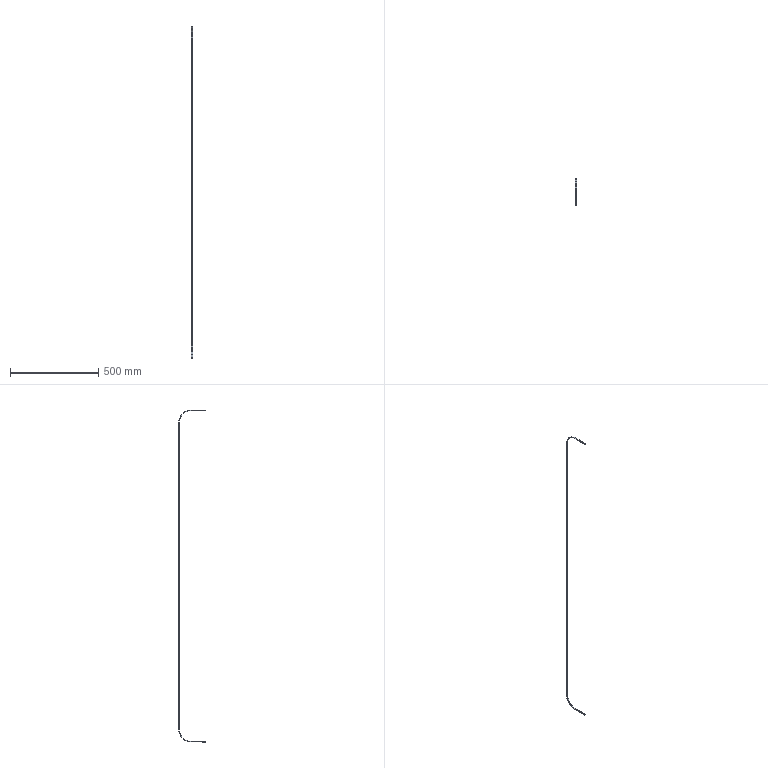Component | SolidWorks | TopHousingAssembly-1_Sealant-2 | 1 solid | 22 faces | box 6 x 149.5 x 1881 mm | volume 38081 mm3 | plane 18 | cylinder 4 | commonest cylinder face diameters 139 x2 133 x2
STEP:
#1=CARTESIAN_POINT('',(43.307,96.791,2.618));
#2=VERTEX_POINT('',#1);
#3=CARTESIAN_POINT('',(43.307,96.909,2.618));
#4=VERTEX_POINT('',#3);
#5=CARTESIAN_POINT('',(43.307,96.909,2.618));
#6=DIRECTION('',(0.,1.,0.));
#7=VECTOR('',#6,39.37);
#8=LINE('',#5,#7);
#9=EDGE_CURVE('',#2,#4,#8,.T.);
#10=ORIENTED_EDGE('',*,*,#9,.F.);
#11=CARTESIAN_POINT('',(43.307,96.791,71.201));
#12=VERTEX_POINT('',#11);
#13=CARTESIAN_POINT('',(43.307,96.791,36.909));
#14=DIRECTION('',(0.,0.,-1.));
#15=VECTOR('',#14,39.37);
#16=LINE('',#13,#15);
#17=EDGE_CURVE('',#12,#2,#16,.T.);
#18=ORIENTED_EDGE('',*,*,#17,.F.);
#19=CARTESIAN_POINT('',(43.307,96.909,71.201));
#20=VERTEX_POINT('',#19);
#21=CARTESIAN_POINT('',(43.307,96.909,71.201));
#22=DIRECTION('',(0.,1.,0.));
#23=VECTOR('',#22,39.37);
#24=LINE('',#21,#23);
#25=EDGE_CURVE('',#12,#20,#24,.T.);
#26=ORIENTED_EDGE('',*,*,#25,.T.);
#27=CARTESIAN_POINT('',(43.307,96.909,71.201));
#28=DIRECTION('',(-0.,0.,-1.));
#29=VECTOR('',#28,39.37);
#30=LINE('',#27,#29);
#31=EDGE_CURVE('',#20,#4,#30,.T.);
#32=ORIENTED_EDGE('',*,*,#31,.T.);
#33=EDGE_LOOP('',(#10,#18,#26,#32));
#34=FACE_OUTER_BOUND('',#33,.T.);
#35=CARTESIAN_POINT('',(43.307,96.909,71.201));
#36=DIRECTION('',(-1.,0.,0.));
#37=DIRECTION('',(-0.,0.,-1.));
#38=AXIS2_PLACEMENT_3D('',#35,#36,#37);
#39=PLANE('',#38);
#40=ADVANCED_FACE('',(#34),#39,.T.);
#41=CARTESIAN_POINT('',(43.543,96.791,71.201));
#42=VERTEX_POINT('',#41);
#43=CARTESIAN_POINT('',(43.543,96.909,71.201));
#44=VERTEX_POINT('',#43);
#45=CARTESIAN_POINT('',(43.543,96.909,71.201));
#46=DIRECTION('',(0.,1.,0.));
#47=VECTOR('',#46,39.37);
#48=LINE('',#45,#47);
#49=EDGE_CURVE('',#42,#44,#48,.T.);
#50=ORIENTED_EDGE('',*,*,#49,.F.);
#51=CARTESIAN_POINT('',(43.543,96.791,2.618));
#52=VERTEX_POINT('',#51);
#53=CARTESIAN_POINT('',(43.543,96.791,36.909));
#54=DIRECTION('',(0.,0.,-1.));
#55=VECTOR('',#54,39.37);
#56=LINE('',#53,#55);
#57=EDGE_CURVE('',#42,#52,#56,.T.);
#58=ORIENTED_EDGE('',*,*,#57,.T.);
#59=CARTESIAN_POINT('',(43.543,96.909,2.618));
#60=VERTEX_POINT('',#59);
#61=CARTESIAN_POINT('',(43.543,96.909,2.618));
#62=DIRECTION('',(0.,1.,0.));
#63=VECTOR('',#62,39.37);
#64=LINE('',#61,#63);
#65=EDGE_CURVE('',#52,#60,#64,.T.);
#66=ORIENTED_EDGE('',*,*,#65,.T.);
#67=CARTESIAN_POINT('',(43.543,96.909,71.201));
#68=DIRECTION('',(-0.,0.,-1.));
#69=VECTOR('',#68,39.37);
#70=LINE('',#67,#69);
#71=EDGE_CURVE('',#44,#60,#70,.T.);
#72=ORIENTED_EDGE('',*,*,#71,.F.);
#73=EDGE_LOOP('',(#50,#58,#66,#72));
#74=FACE_OUTER_BOUND('',#73,.T.);
#75=CARTESIAN_POINT('',(43.543,96.909,71.201));
#76=DIRECTION('',(-1.,0.,0.));
#77=DIRECTION('',(-0.,0.,-1.));
#78=AXIS2_PLACEMENT_3D('',#75,#76,#77);
#79=PLANE('',#78);
#80=ADVANCED_FACE('',(#74),#79,.F.);
#81=ORIENTED_EDGE('',*,*,#71,.T.);
#82=CARTESIAN_POINT('',(43.307,96.909,2.618));
#83=DIRECTION('',(1.,0.,0.));
#84=VECTOR('',#83,39.37);
#85=LINE('',#82,#84);
#86=EDGE_CURVE('',#4,#60,#85,.T.);
#87=ORIENTED_EDGE('',*,*,#86,.F.);
#88=ORIENTED_EDGE('',*,*,#31,.F.);
#89=CARTESIAN_POINT('',(43.543,96.909,71.201));
#90=DIRECTION('',(-1.,0.,0.));
#91=VECTOR('',#90,39.37);
#92=LINE('',#89,#91);
#93=EDGE_CURVE('',#44,#20,#92,.T.);
#94=ORIENTED_EDGE('',*,*,#93,.F.);
#95=EDGE_LOOP('',(#81,#87,#88,#94));
#96=FACE_OUTER_BOUND('',#95,.T.);
#97=CARTESIAN_POINT('',(43.425,96.909,36.909));
#98=DIRECTION('',(0.,-1.,0.));
#99=DIRECTION('',(-1.,0.,0.));
#100=AXIS2_PLACEMENT_3D('',#97,#98,#99);
#101=PLANE('',#100);
#102=ADVANCED_FACE('',(#96),#101,.F.);
#103=ORIENTED_EDGE('',*,*,#57,.F.);
#104=CARTESIAN_POINT('',(43.425,96.791,71.201));
#105=DIRECTION('',(-1.,0.,0.));
#106=VECTOR('',#105,39.37);
#107=LINE('',#104,#106);
#108=EDGE_CURVE('',#42,#12,#107,.T.);
#109=ORIENTED_EDGE('',*,*,#108,.T.);
#110=ORIENTED_EDGE('',*,*,#17,.T.);
#111=CARTESIAN_POINT('',(43.425,96.791,2.618));
#112=DIRECTION('',(1.,0.,0.));
#113=VECTOR('',#112,39.37);
#114=LINE('',#111,#113);
#115=EDGE_CURVE('',#2,#52,#114,.T.);
#116=ORIENTED_EDGE('',*,*,#115,.T.);
#117=EDGE_LOOP('',(#103,#109,#110,#116));
#118=FACE_OUTER_BOUND('',#117,.T.);
#119=CARTESIAN_POINT('',(43.425,96.791,36.909));
#120=DIRECTION('',(0.,-1.,0.));
#121=DIRECTION('',(-1.,0.,0.));
#122=AXIS2_PLACEMENT_3D('',#119,#120,#121);
#123=PLANE('',#122);
#124=ADVANCED_FACE('',(#118),#123,.T.);
#125=CARTESIAN_POINT('',(43.543,94.173,73.819));
#126=VERTEX_POINT('',#125);
#127=CARTESIAN_POINT('',(43.543,94.173,73.937));
#128=VERTEX_POINT('',#127);
#129=CARTESIAN_POINT('',(43.543,94.173,73.937));
#130=DIRECTION('',(0.,0.,1.));
#131=VECTOR('',#130,39.37);
#132=LINE('',#129,#131);
#133=EDGE_CURVE('',#126,#128,#132,.T.);
#134=ORIENTED_EDGE('',*,*,#133,.F.);
#135=CARTESIAN_POINT('',(43.543,94.173,71.201));
#136=DIRECTION('',(1.,0.,0.));
#137=DIRECTION('',(0.,-0.,1.));
#138=AXIS2_PLACEMENT_3D('',#135,#136,#137);
#139=CIRCLE('',#138,2.618);
#140=EDGE_CURVE('',#42,#126,#139,.T.);
#141=ORIENTED_EDGE('',*,*,#140,.F.);
#142=ORIENTED_EDGE('',*,*,#49,.T.);
#143=CARTESIAN_POINT('',(43.543,94.173,71.201));
#144=DIRECTION('',(1.,0.,0.));
#145=DIRECTION('',(0.,-0.,1.));
#146=AXIS2_PLACEMENT_3D('',#143,#144,#145);
#147=CIRCLE('',#146,2.736);
#148=EDGE_CURVE('',#44,#128,#147,.T.);
#149=ORIENTED_EDGE('',*,*,#148,.T.);
#150=EDGE_LOOP('',(#134,#141,#142,#149));
#151=FACE_OUTER_BOUND('',#150,.T.);
#152=CARTESIAN_POINT('',(43.543,94.173,71.201));
#153=DIRECTION('',(1.,0.,0.));
#154=DIRECTION('',(0.,0.,-1.));
#155=AXIS2_PLACEMENT_3D('',#152,#153,#154);
#156=PLANE('',#155);
#157=ADVANCED_FACE('',(#151),#156,.T.);
#158=CARTESIAN_POINT('',(43.307,94.173,73.819));
#159=VERTEX_POINT('',#158);
#160=CARTESIAN_POINT('',(43.307,94.173,71.201));
#161=DIRECTION('',(-1.,0.,0.));
#162=DIRECTION('',(0.,0.,1.));
#163=AXIS2_PLACEMENT_3D('',#160,#161,#162);
#164=CIRCLE('',#163,2.618);
#165=EDGE_CURVE('',#159,#12,#164,.T.);
#166=ORIENTED_EDGE('',*,*,#165,.F.);
#167=CARTESIAN_POINT('',(43.307,94.173,73.937));
#168=VERTEX_POINT('',#167);
#169=CARTESIAN_POINT('',(43.307,94.173,73.819));
#170=DIRECTION('',(0.,0.,1.));
#171=VECTOR('',#170,39.37);
#172=LINE('',#169,#171);
#173=EDGE_CURVE('',#159,#168,#172,.T.);
#174=ORIENTED_EDGE('',*,*,#173,.T.);
#175=CARTESIAN_POINT('',(43.307,94.173,71.201));
#176=DIRECTION('',(-1.,0.,0.));
#177=DIRECTION('',(0.,0.,1.));
#178=AXIS2_PLACEMENT_3D('',#175,#176,#177);
#179=CIRCLE('',#178,2.736);
#180=EDGE_CURVE('',#168,#20,#179,.T.);
#181=ORIENTED_EDGE('',*,*,#180,.T.);
#182=ORIENTED_EDGE('',*,*,#25,.F.);
#183=EDGE_LOOP('',(#166,#174,#181,#182));
#184=FACE_OUTER_BOUND('',#183,.T.);
#185=CARTESIAN_POINT('',(43.307,94.173,71.201));
#186=DIRECTION('',(1.,0.,0.));
#187=DIRECTION('',(0.,0.,-1.));
#188=AXIS2_PLACEMENT_3D('',#185,#186,#187);
#189=PLANE('',#188);
#190=ADVANCED_FACE('',(#184),#189,.F.);
#191=ORIENTED_EDGE('',*,*,#93,.T.);
#192=ORIENTED_EDGE('',*,*,#180,.F.);
#193=CARTESIAN_POINT('',(43.543,94.173,73.937));
#194=DIRECTION('',(1.,0.,0.));
#195=VECTOR('',#194,39.37);
#196=LINE('',#193,#195);
#197=EDGE_CURVE('',#168,#128,#196,.T.);
#198=ORIENTED_EDGE('',*,*,#197,.T.);
#199=ORIENTED_EDGE('',*,*,#148,.F.);
#200=EDGE_LOOP('',(#191,#192,#198,#199));
#201=FACE_OUTER_BOUND('',#200,.T.);
#202=CARTESIAN_POINT('',(43.307,94.173,71.201));
#203=DIRECTION('',(-1.,0.,0.));
#204=DIRECTION('',(0.,0.,1.));
#205=AXIS2_PLACEMENT_3D('',#202,#203,#204);
#206=CYLINDRICAL_SURFACE('',#205,2.736);
#207=ADVANCED_FACE('',(#201),#206,.T.);
#208=ORIENTED_EDGE('',*,*,#108,.F.);
#209=ORIENTED_EDGE('',*,*,#140,.T.);
#210=CARTESIAN_POINT('',(43.543,94.173,73.819));
#211=DIRECTION('',(-1.,0.,0.));
#212=VECTOR('',#211,39.37);
#213=LINE('',#210,#212);
#214=EDGE_CURVE('',#126,#159,#213,.T.);
#215=ORIENTED_EDGE('',*,*,#214,.T.);
#216=ORIENTED_EDGE('',*,*,#165,.T.);
#217=EDGE_LOOP('',(#208,#209,#215,#216));
#218=FACE_OUTER_BOUND('',#217,.T.);
#219=CARTESIAN_POINT('',(43.307,94.173,71.201));
#220=DIRECTION('',(-1.,0.,0.));
#221=DIRECTION('',(0.,0.,1.));
#222=AXIS2_PLACEMENT_3D('',#219,#220,#221);
#223=CYLINDRICAL_SURFACE('',#222,2.618);
#224=ADVANCED_FACE('',(#218),#223,.F.);
#225=ORIENTED_EDGE('',*,*,#133,.T.);
#226=CARTESIAN_POINT('',(43.543,91.024,73.937));
#227=VERTEX_POINT('',#226);
#228=CARTESIAN_POINT('',(43.543,96.791,73.937));
#229=DIRECTION('',(0.,1.,-0.));
#230=VECTOR('',#229,39.37);
#231=LINE('',#228,#230);
#232=EDGE_CURVE('',#227,#128,#231,.T.);
#233=ORIENTED_EDGE('',*,*,#232,.F.);
#234=CARTESIAN_POINT('',(43.543,91.024,73.819));
#235=VERTEX_POINT('',#234);
#236=CARTESIAN_POINT('',(43.543,91.024,73.937));
#237=DIRECTION('',(0.,-0.,-1.));
#238=VECTOR('',#237,39.37);
#239=LINE('',#236,#238);
#240=EDGE_CURVE('',#227,#235,#239,.T.);
#241=ORIENTED_EDGE('',*,*,#240,.T.);
#242=CARTESIAN_POINT('',(43.543,96.791,73.819));
#243=DIRECTION('',(0.,1.,-0.));
#244=VECTOR('',#243,39.37);
#245=LINE('',#242,#244);
#246=EDGE_CURVE('',#235,#126,#245,.T.);
#247=ORIENTED_EDGE('',*,*,#246,.T.);
#248=EDGE_LOOP('',(#225,#233,#241,#247));
#249=FACE_OUTER_BOUND('',#248,.T.);
#250=CARTESIAN_POINT('',(43.543,96.791,73.937));
#251=DIRECTION('',(-1.,0.,0.));
#252=DIRECTION('',(0.,0.,1.));
#253=AXIS2_PLACEMENT_3D('',#250,#251,#252);
#254=PLANE('',#253);
#255=ADVANCED_FACE('',(#249),#254,.F.);
#256=ORIENTED_EDGE('',*,*,#173,.F.);
#257=CARTESIAN_POINT('',(43.307,91.024,73.819));
#258=VERTEX_POINT('',#257);
#259=CARTESIAN_POINT('',(43.307,91.024,73.819));
#260=DIRECTION('',(0.,-1.,0.));
#261=VECTOR('',#260,39.37);
#262=LINE('',#259,#261);
#263=EDGE_CURVE('',#159,#258,#262,.T.);
#264=ORIENTED_EDGE('',*,*,#263,.T.);
#265=CARTESIAN_POINT('',(43.307,91.024,73.937));
#266=VERTEX_POINT('',#265);
#267=CARTESIAN_POINT('',(43.307,91.024,73.937));
#268=DIRECTION('',(0.,-0.,-1.));
#269=VECTOR('',#268,39.37);
#270=LINE('',#267,#269);
#271=EDGE_CURVE('',#266,#258,#270,.T.);
#272=ORIENTED_EDGE('',*,*,#271,.F.);
#273=CARTESIAN_POINT('',(43.307,96.791,73.937));
#274=DIRECTION('',(0.,-1.,0.));
#275=VECTOR('',#274,39.37);
#276=LINE('',#273,#275);
#277=EDGE_CURVE('',#168,#266,#276,.T.);
#278=ORIENTED_EDGE('',*,*,#277,.F.);
#279=EDGE_LOOP('',(#256,#264,#272,#278));
#280=FACE_OUTER_BOUND('',#279,.T.);
#281=CARTESIAN_POINT('',(43.307,91.024,73.937));
#282=DIRECTION('',(1.,0.,0.));
#283=DIRECTION('',(0.,0.,-1.));
#284=AXIS2_PLACEMENT_3D('',#281,#282,#283);
#285=PLANE('',#284);
#286=ADVANCED_FACE('',(#280),#285,.F.);
#287=ORIENTED_EDGE('',*,*,#197,.F.);
#288=ORIENTED_EDGE('',*,*,#277,.T.);
#289=CARTESIAN_POINT('',(43.425,91.024,73.937));
#290=DIRECTION('',(1.,0.,0.));
#291=VECTOR('',#290,39.37);
#292=LINE('',#289,#291);
#293=EDGE_CURVE('',#266,#227,#292,.T.);
#294=ORIENTED_EDGE('',*,*,#293,.T.);
#295=ORIENTED_EDGE('',*,*,#232,.T.);
#296=EDGE_LOOP('',(#287,#288,#294,#295));
#297=FACE_OUTER_BOUND('',#296,.T.);
#298=CARTESIAN_POINT('',(43.425,96.791,73.937));
#299=DIRECTION('',(0.,-0.,-1.));
#300=DIRECTION('',(0.,1.,-0.));
#301=AXIS2_PLACEMENT_3D('',#298,#299,#300);
#302=PLANE('',#301);
#303=ADVANCED_FACE('',(#297),#302,.F.);
#304=ORIENTED_EDGE('',*,*,#263,.F.);
#305=ORIENTED_EDGE('',*,*,#214,.F.);
#306=ORIENTED_EDGE('',*,*,#246,.F.);
#307=CARTESIAN_POINT('',(43.543,91.024,73.819));
#308=DIRECTION('',(1.,0.,0.));
#309=VECTOR('',#308,39.37);
#310=LINE('',#307,#309);
#311=EDGE_CURVE('',#258,#235,#310,.T.);
#312=ORIENTED_EDGE('',*,*,#311,.F.);
#313=EDGE_LOOP('',(#304,#305,#306,#312));
#314=FACE_OUTER_BOUND('',#313,.T.);
#315=CARTESIAN_POINT('',(43.425,96.791,73.819));
#316=DIRECTION('',(0.,-0.,-1.));
#317=DIRECTION('',(0.,1.,-0.));
#318=AXIS2_PLACEMENT_3D('',#315,#316,#317);
#319=PLANE('',#318);
#320=ADVANCED_FACE('',(#314),#319,.T.);
#321=ORIENTED_EDGE('',*,*,#311,.T.);
#322=ORIENTED_EDGE('',*,*,#240,.F.);
#323=ORIENTED_EDGE('',*,*,#293,.F.);
#324=ORIENTED_EDGE('',*,*,#271,.T.);
#325=EDGE_LOOP('',(#321,#322,#323,#324));
#326=FACE_OUTER_BOUND('',#325,.T.);
#327=CARTESIAN_POINT('',(43.543,91.024,73.937));
#328=DIRECTION('',(0.,1.,-0.));
#329=DIRECTION('',(0.,0.,1.));
#330=AXIS2_PLACEMENT_3D('',#327,#328,#329);
#331=PLANE('',#330);
#332=ADVANCED_FACE('',(#326),#331,.F.);
#333=CARTESIAN_POINT('',(43.307,94.173,-0.));
#334=VERTEX_POINT('',#333);
#335=CARTESIAN_POINT('',(43.307,94.173,-0.1181));
#336=VERTEX_POINT('',#335);
#337=CARTESIAN_POINT('',(43.307,94.173,-0.1181));
#338=DIRECTION('',(0.,0.,-1.));
#339=VECTOR('',#338,39.37);
#340=LINE('',#337,#339);
#341=EDGE_CURVE('',#334,#336,#340,.T.);
#342=ORIENTED_EDGE('',*,*,#341,.F.);
#343=CARTESIAN_POINT('',(43.307,94.173,2.618));
#344=DIRECTION('',(-1.,0.,0.));
#345=DIRECTION('',(0.,-0.,-1.));
#346=AXIS2_PLACEMENT_3D('',#343,#344,#345);
#347=CIRCLE('',#346,2.618);
#348=EDGE_CURVE('',#2,#334,#347,.T.);
#349=ORIENTED_EDGE('',*,*,#348,.F.);
#350=ORIENTED_EDGE('',*,*,#9,.T.);
#351=CARTESIAN_POINT('',(43.307,94.173,2.618));
#352=DIRECTION('',(-1.,0.,0.));
#353=DIRECTION('',(0.,-0.,-1.));
#354=AXIS2_PLACEMENT_3D('',#351,#352,#353);
#355=CIRCLE('',#354,2.736);
#356=EDGE_CURVE('',#4,#336,#355,.T.);
#357=ORIENTED_EDGE('',*,*,#356,.T.);
#358=EDGE_LOOP('',(#342,#349,#350,#357));
#359=FACE_OUTER_BOUND('',#358,.T.);
#360=CARTESIAN_POINT('',(43.307,94.173,2.618));
#361=DIRECTION('',(-1.,0.,0.));
#362=DIRECTION('',(0.,0.,1.));
#363=AXIS2_PLACEMENT_3D('',#360,#361,#362);
#364=PLANE('',#363);
#365=ADVANCED_FACE('',(#359),#364,.T.);
#366=CARTESIAN_POINT('',(43.543,94.173,-0.));
#367=VERTEX_POINT('',#366);
#368=CARTESIAN_POINT('',(43.543,94.173,2.618));
#369=DIRECTION('',(1.,0.,0.));
#370=DIRECTION('',(0.,0.,-1.));
#371=AXIS2_PLACEMENT_3D('',#368,#369,#370);
#372=CIRCLE('',#371,2.618);
#373=EDGE_CURVE('',#367,#52,#372,.T.);
#374=ORIENTED_EDGE('',*,*,#373,.F.);
#375=CARTESIAN_POINT('',(43.543,94.173,-0.1181));
#376=VERTEX_POINT('',#375);
#377=CARTESIAN_POINT('',(43.543,94.173,-0.));
#378=DIRECTION('',(0.,0.,-1.));
#379=VECTOR('',#378,39.37);
#380=LINE('',#377,#379);
#381=EDGE_CURVE('',#367,#376,#380,.T.);
#382=ORIENTED_EDGE('',*,*,#381,.T.);
#383=CARTESIAN_POINT('',(43.543,94.173,2.618));
#384=DIRECTION('',(1.,0.,0.));
#385=DIRECTION('',(0.,0.,-1.));
#386=AXIS2_PLACEMENT_3D('',#383,#384,#385);
#387=CIRCLE('',#386,2.736);
#388=EDGE_CURVE('',#376,#60,#387,.T.);
#389=ORIENTED_EDGE('',*,*,#388,.T.);
#390=ORIENTED_EDGE('',*,*,#65,.F.);
#391=EDGE_LOOP('',(#374,#382,#389,#390));
#392=FACE_OUTER_BOUND('',#391,.T.);
#393=CARTESIAN_POINT('',(43.543,94.173,2.618));
#394=DIRECTION('',(-1.,0.,0.));
#395=DIRECTION('',(0.,0.,1.));
#396=AXIS2_PLACEMENT_3D('',#393,#394,#395);
#397=PLANE('',#396);
#398=ADVANCED_FACE('',(#392),#397,.F.);
#399=ORIENTED_EDGE('',*,*,#86,.T.);
#400=ORIENTED_EDGE('',*,*,#388,.F.);
#401=CARTESIAN_POINT('',(43.307,94.173,-0.1181));
#402=DIRECTION('',(-1.,0.,0.));
#403=VECTOR('',#402,39.37);
#404=LINE('',#401,#403);
#405=EDGE_CURVE('',#376,#336,#404,.T.);
#406=ORIENTED_EDGE('',*,*,#405,.T.);
#407=ORIENTED_EDGE('',*,*,#356,.F.);
#408=EDGE_LOOP('',(#399,#400,#406,#407));
#409=FACE_OUTER_BOUND('',#408,.T.);
#410=CARTESIAN_POINT('',(43.543,94.173,2.618));
#411=DIRECTION('',(1.,0.,0.));
#412=DIRECTION('',(0.,0.,-1.));
#413=AXIS2_PLACEMENT_3D('',#410,#411,#412);
#414=CYLINDRICAL_SURFACE('',#413,2.736);
#415=ADVANCED_FACE('',(#409),#414,.T.);
#416=ORIENTED_EDGE('',*,*,#115,.F.);
#417=ORIENTED_EDGE('',*,*,#348,.T.);
#418=CARTESIAN_POINT('',(43.307,94.173,-0.));
#419=DIRECTION('',(1.,0.,0.));
#420=VECTOR('',#419,39.37);
#421=LINE('',#418,#420);
#422=EDGE_CURVE('',#334,#367,#421,.T.);
#423=ORIENTED_EDGE('',*,*,#422,.T.);
#424=ORIENTED_EDGE('',*,*,#373,.T.);
#425=EDGE_LOOP('',(#416,#417,#423,#424));
#426=FACE_OUTER_BOUND('',#425,.T.);
#427=CARTESIAN_POINT('',(43.543,94.173,2.618));
#428=DIRECTION('',(1.,0.,0.));
#429=DIRECTION('',(0.,0.,-1.));
#430=AXIS2_PLACEMENT_3D('',#427,#428,#429);
#431=CYLINDRICAL_SURFACE('',#430,2.618);
#432=ADVANCED_FACE('',(#426),#431,.F.);
#433=ORIENTED_EDGE('',*,*,#341,.T.);
#434=CARTESIAN_POINT('',(43.307,91.024,-0.1181));
#435=VERTEX_POINT('',#434);
#436=CARTESIAN_POINT('',(43.307,96.791,-0.1181));
#437=DIRECTION('',(0.,1.,0.));
#438=VECTOR('',#437,39.37);
#439=LINE('',#436,#438);
#440=EDGE_CURVE('',#435,#336,#439,.T.);
#441=ORIENTED_EDGE('',*,*,#440,.F.);
#442=CARTESIAN_POINT('',(43.307,91.024,-0.));
#443=VERTEX_POINT('',#442);
#444=CARTESIAN_POINT('',(43.307,91.024,-0.1181));
#445=DIRECTION('',(0.,-0.,1.));
#446=VECTOR('',#445,39.37);
#447=LINE('',#444,#446);
#448=EDGE_CURVE('',#435,#443,#447,.T.);
#449=ORIENTED_EDGE('',*,*,#448,.T.);
#450=CARTESIAN_POINT('',(43.307,96.791,-0.));
#451=DIRECTION('',(0.,1.,0.));
#452=VECTOR('',#451,39.37);
#453=LINE('',#450,#452);
#454=EDGE_CURVE('',#443,#334,#453,.T.);
#455=ORIENTED_EDGE('',*,*,#454,.T.);
#456=EDGE_LOOP('',(#433,#441,#449,#455));
#457=FACE_OUTER_BOUND('',#456,.T.);
#458=CARTESIAN_POINT('',(43.307,96.791,-0.1181));
#459=DIRECTION('',(1.,0.,0.));
#460=DIRECTION('',(0.,0.,-1.));
#461=AXIS2_PLACEMENT_3D('',#458,#459,#460);
#462=PLANE('',#461);
#463=ADVANCED_FACE('',(#457),#462,.F.);
#464=ORIENTED_EDGE('',*,*,#381,.F.);
#465=CARTESIAN_POINT('',(43.543,91.024,-0.));
#466=VERTEX_POINT('',#465);
#467=CARTESIAN_POINT('',(43.543,91.024,-0.));
#468=DIRECTION('',(0.,-1.,-0.));
#469=VECTOR('',#468,39.37);
#470=LINE('',#467,#469);
#471=EDGE_CURVE('',#367,#466,#470,.T.);
#472=ORIENTED_EDGE('',*,*,#471,.T.);
#473=CARTESIAN_POINT('',(43.543,91.024,-0.1181));
#474=VERTEX_POINT('',#473);
#475=CARTESIAN_POINT('',(43.543,91.024,-0.1181));
#476=DIRECTION('',(0.,-0.,1.));
#477=VECTOR('',#476,39.37);
#478=LINE('',#475,#477);
#479=EDGE_CURVE('',#474,#466,#478,.T.);
#480=ORIENTED_EDGE('',*,*,#479,.F.);
#481=CARTESIAN_POINT('',(43.543,96.791,-0.1181));
#482=DIRECTION('',(0.,-1.,-0.));
#483=VECTOR('',#482,39.37);
#484=LINE('',#481,#483);
#485=EDGE_CURVE('',#376,#474,#484,.T.);
#486=ORIENTED_EDGE('',*,*,#485,.F.);
#487=EDGE_LOOP('',(#464,#472,#480,#486));
#488=FACE_OUTER_BOUND('',#487,.T.);
#489=CARTESIAN_POINT('',(43.543,91.024,-0.1181));
#490=DIRECTION('',(-1.,0.,0.));
#491=DIRECTION('',(0.,0.,1.));
#492=AXIS2_PLACEMENT_3D('',#489,#490,#491);
#493=PLANE('',#492);
#494=ADVANCED_FACE('',(#488),#493,.F.);
#495=ORIENTED_EDGE('',*,*,#405,.F.);
#496=ORIENTED_EDGE('',*,*,#485,.T.);
#497=CARTESIAN_POINT('',(43.425,91.024,-0.1181));
#498=DIRECTION('',(-1.,0.,0.));
#499=VECTOR('',#498,39.37);
#500=LINE('',#497,#499);
#501=EDGE_CURVE('',#474,#435,#500,.T.);
#502=ORIENTED_EDGE('',*,*,#501,.T.);
#503=ORIENTED_EDGE('',*,*,#440,.T.);
#504=EDGE_LOOP('',(#495,#496,#502,#503));
#505=FACE_OUTER_BOUND('',#504,.T.);
#506=CARTESIAN_POINT('',(43.425,96.791,-0.1181));
#507=DIRECTION('',(0.,-0.,1.));
#508=DIRECTION('',(0.,-1.,-0.));
#509=AXIS2_PLACEMENT_3D('',#506,#507,#508);
#510=PLANE('',#509);
#511=ADVANCED_FACE('',(#505),#510,.F.);
#512=ORIENTED_EDGE('',*,*,#471,.F.);
#513=ORIENTED_EDGE('',*,*,#422,.F.);
#514=ORIENTED_EDGE('',*,*,#454,.F.);
#515=CARTESIAN_POINT('',(43.307,91.024,-0.));
#516=DIRECTION('',(-1.,0.,0.));
#517=VECTOR('',#516,39.37);
#518=LINE('',#515,#517);
#519=EDGE_CURVE('',#466,#443,#518,.T.);
#520=ORIENTED_EDGE('',*,*,#519,.F.);
#521=EDGE_LOOP('',(#512,#513,#514,#520));
#522=FACE_OUTER_BOUND('',#521,.T.);
#523=CARTESIAN_POINT('',(43.425,96.791,-0.));
#524=DIRECTION('',(0.,-0.,1.));
#525=DIRECTION('',(0.,-1.,-0.));
#526=AXIS2_PLACEMENT_3D('',#523,#524,#525);
#527=PLANE('',#526);
#528=ADVANCED_FACE('',(#522),#527,.T.);
#529=ORIENTED_EDGE('',*,*,#519,.T.);
#530=ORIENTED_EDGE('',*,*,#448,.F.);
#531=ORIENTED_EDGE('',*,*,#501,.F.);
#532=ORIENTED_EDGE('',*,*,#479,.T.);
#533=EDGE_LOOP('',(#529,#530,#531,#532));
#534=FACE_OUTER_BOUND('',#533,.T.);
#535=CARTESIAN_POINT('',(43.307,91.024,-0.1181));
#536=DIRECTION('',(0.,1.,0.));
#537=DIRECTION('',(0.,-0.,1.));
#538=AXIS2_PLACEMENT_3D('',#535,#536,#537);
#539=PLANE('',#538);
#540=ADVANCED_FACE('',(#534),#539,.F.);
#541=CLOSED_SHELL('',(#40,#80,#102,#124,#157,#190,#207,#224,#255,#286,#303,#320,#332,#365,#398,#415,#432,#463,#494,#511,#528,#540));
#542=MANIFOLD_SOLID_BREP('',#541);
#543=CARTESIAN_POINT('',(0.,0.,0.));
#544=DIRECTION('',(0.,0.,1.));
#545=DIRECTION('',(1.,0.,0.));
#546=AXIS2_PLACEMENT_3D('',#543,#544,#545);
#547=(LENGTH_UNIT()NAMED_UNIT(*)SI_UNIT($,.METRE.));
#548=LENGTH_MEASURE_WITH_UNIT(LENGTH_MEASURE(0.0254),#547);
#549=DIMENSIONAL_EXPONENTS(1.,0.,0.,0.,0.,0.,0.);
#550=(CONVERSION_BASED_UNIT('',#548)LENGTH_UNIT()NAMED_UNIT(#549));
#551=UNCERTAINTY_MEASURE_WITH_UNIT(LENGTH_MEASURE(0.00001),#550,'','');
#552=(NAMED_UNIT(*)PLANE_ANGLE_UNIT()SI_UNIT($,.RADIAN.));
#553=(NAMED_UNIT(*)SI_UNIT($,.STERADIAN.)SOLID_ANGLE_UNIT());
#554=(GEOMETRIC_REPRESENTATION_CONTEXT(3)GLOBAL_UNCERTAINTY_ASSIGNED_CONTEXT((#551))GLOBAL_UNIT_ASSIGNED_CONTEXT((#550,#552,#553))REPRESENTATION_CONTEXT('',''));
#555=ADVANCED_BREP_SHAPE_REPRESENTATION('',(#542,#546),#554);
#556=COLOUR_RGB('',0.7922,0.8196,0.9333);
#557=FILL_AREA_STYLE_COLOUR('',#556);
#558=FILL_AREA_STYLE('',(#557));
#559=SURFACE_STYLE_FILL_AREA(#558);
#560=SURFACE_SIDE_STYLE('',(#559));
#561=SURFACE_STYLE_USAGE(.BOTH.,#560);
#562=PRESENTATION_STYLE_ASSIGNMENT((#561));
#563=STYLED_ITEM('',(#562),#542);
#564=PRESENTATION_LAYER_ASSIGNMENT('','',(#563));
#565=(LENGTH_UNIT()NAMED_UNIT(*)SI_UNIT($,.METRE.));
#566=LENGTH_MEASURE_WITH_UNIT(LENGTH_MEASURE(0.0254),#565);
#567=DIMENSIONAL_EXPONENTS(1.,0.,0.,0.,0.,0.,0.);
#568=(CONVERSION_BASED_UNIT('',#566)LENGTH_UNIT()NAMED_UNIT(#567));
#569=UNCERTAINTY_MEASURE_WITH_UNIT(LENGTH_MEASURE(0.00001),#568,'','');
#570=(NAMED_UNIT(*)PLANE_ANGLE_UNIT()SI_UNIT($,.RADIAN.));
#571=(NAMED_UNIT(*)SI_UNIT($,.STERADIAN.)SOLID_ANGLE_UNIT());
#572=(GEOMETRIC_REPRESENTATION_CONTEXT(3)GLOBAL_UNCERTAINTY_ASSIGNED_CONTEXT((#569))GLOBAL_UNIT_ASSIGNED_CONTEXT((#568,#570,#571))REPRESENTATION_CONTEXT('',''));
#573=MECHANICAL_DESIGN_GEOMETRIC_PRESENTATION_REPRESENTATION('',(#563),#572);